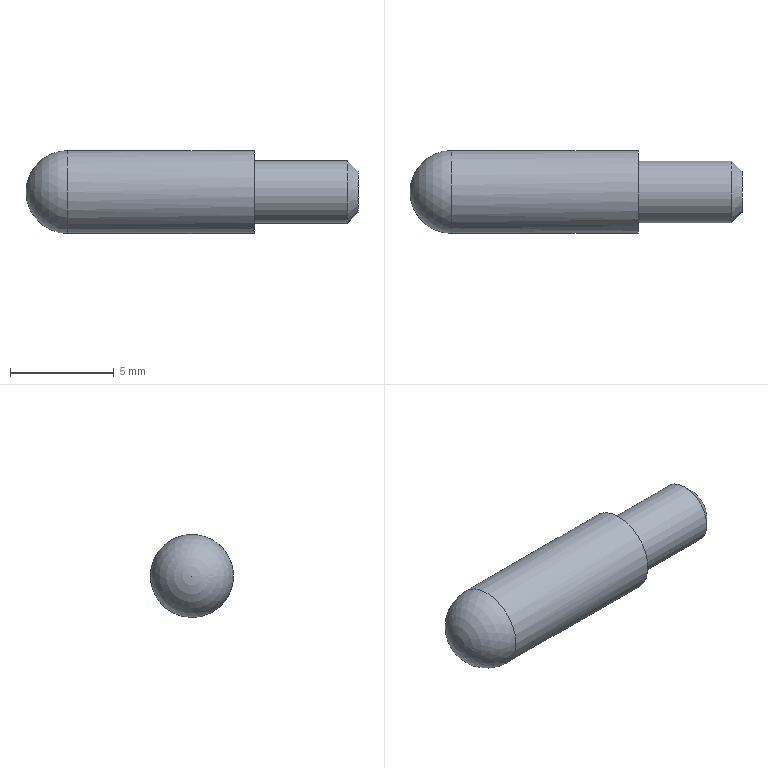Component | NX | ASSY_PRAC_PART_7 | 1 solid | 6 faces | box 16 x 4 x 4 mm | volume 164 mm3 | cylinder 2 | plane 2 | sphere 1 | cone 1 | commonest cylinder face diameters 4 x1 3 x1
STEP:
#1=CARTESIAN_POINT('',(0.,0.,0.));
#2=DIRECTION('',(0.,0.,1.));
#3=DIRECTION('',(1.,0.,0.));
#4=AXIS2_PLACEMENT_3D('',#1,#2,#3);
#5=CARTESIAN_POINT('',(-22.5,0.3851,13.561));
#6=VERTEX_POINT('',#5);
#7=CARTESIAN_POINT('',(-22.5,-1.615,15.561));
#8=VERTEX_POINT('',#7);
#9=CARTESIAN_POINT('',(-22.5,0.3851,15.561));
#10=DIRECTION('',(-1.,0.,0.));
#11=DIRECTION('',(0.,0.,-1.));
#12=AXIS2_PLACEMENT_3D('',#9,#10,#11);
#13=CIRCLE('',#12,2.);
#14=CARTESIAN_POINT('',(-22.5,0.3851,15.561));
#15=DIRECTION('',(-1.,-0.,0.));
#16=DIRECTION('',(0.,-1.,0.));
#17=AXIS2_PLACEMENT_3D('',#14,#15,#16);
#18=SPHERICAL_SURFACE('',#17,2.);
#19=CARTESIAN_POINT('',(4.712,0.));
#20=CARTESIAN_POINT('',(4.808,0.));
#21=CARTESIAN_POINT('',(4.998,0.));
#22=CARTESIAN_POINT('',(5.284,0.));
#23=CARTESIAN_POINT('',(5.569,0.));
#24=CARTESIAN_POINT('',(5.855,0.));
#25=CARTESIAN_POINT('',(6.14,0.));
#26=CARTESIAN_POINT('',(6.426,0.));
#27=CARTESIAN_POINT('',(6.712,0.));
#28=CARTESIAN_POINT('',(6.997,0.));
#29=CARTESIAN_POINT('',(7.283,0.));
#30=CARTESIAN_POINT('',(7.568,0.));
#31=CARTESIAN_POINT('',(7.854,0.));
#32=CARTESIAN_POINT('',(8.14,0.));
#33=CARTESIAN_POINT('',(8.425,0.));
#34=CARTESIAN_POINT('',(8.711,0.));
#35=CARTESIAN_POINT('',(8.996,0.));
#36=CARTESIAN_POINT('',(9.282,0.));
#37=CARTESIAN_POINT('',(9.568,0.));
#38=CARTESIAN_POINT('',(9.853,0.));
#39=CARTESIAN_POINT('',(10.139,0.));
#40=CARTESIAN_POINT('',(10.424,0.));
#41=CARTESIAN_POINT('',(10.71,0.));
#42=CARTESIAN_POINT('',(10.9,0.));
#43=CARTESIAN_POINT('',(10.996,0.));
#44=B_SPLINE_CURVE_WITH_KNOTS('',3,(#19,#20,#21,#22,#23,#24,#25,#26,#27,#28,#29,#30,#31,#32,#33,#34,#35,#36,#37,#38,#39,#40,#41,#42,#43),.UNSPECIFIED.,.F.,.F.,(4,1,1,1,1,1,1,1,1,1,1,1,1,1,1,1,1,1,1,1,1,1,4),(0.,0.2856,0.5712,0.8568,1.142,1.428,1.714,1.999,2.285,2.57,2.856,3.142,3.427,3.713,3.998,4.284,4.57,4.855,5.141,5.426,5.712,5.998,6.283),.QUASI_UNIFORM_KNOTS.);
#45=(GEOMETRIC_REPRESENTATION_CONTEXT(2)PARAMETRIC_REPRESENTATION_CONTEXT()REPRESENTATION_CONTEXT('',''));
#46=DEFINITIONAL_REPRESENTATION('',(#44),#45);
#47=PCURVE('',#18,#46);
#48=CARTESIAN_POINT('',(-24.5,0.3851,15.561));
#49=DIRECTION('',(-1.,0.,0.));
#50=DIRECTION('',(0.,0.,-1.));
#51=AXIS2_PLACEMENT_3D('',#48,#49,#50);
#52=CYLINDRICAL_SURFACE('',#51,2.);
#53=CARTESIAN_POINT('',(0.,-2.));
#54=DIRECTION('',(1.,0.));
#55=VECTOR('',#54,1.);
#56=LINE('',#53,#55);
#57=(GEOMETRIC_REPRESENTATION_CONTEXT(2)PARAMETRIC_REPRESENTATION_CONTEXT()REPRESENTATION_CONTEXT('',''));
#58=DEFINITIONAL_REPRESENTATION('',(#56),#57);
#59=PCURVE('',#52,#58);
#60=SURFACE_CURVE('',#13,(#47,#59),.PCURVE_S1.);
#61=EDGE_CURVE('',#6,#8,#60,.T.);
#62=ORIENTED_EDGE('',*,*,#61,.T.);
#63=CARTESIAN_POINT('',(-24.5,0.3851,15.561));
#64=VERTEX_POINT('',#63);
#65=CARTESIAN_POINT('',(-22.5,-1.615,15.561));
#66=CARTESIAN_POINT('',(-23.024,-1.615,15.561));
#67=CARTESIAN_POINT('',(-23.547,-1.45,15.561));
#68=CARTESIAN_POINT('',(-24.006,-1.121,15.561));
#69=CARTESIAN_POINT('',(-24.336,-0.6621,15.561));
#70=CARTESIAN_POINT('',(-24.5,-0.1385,15.561));
#71=CARTESIAN_POINT('',(-24.5,0.3851,15.561));
#72=B_SPLINE_CURVE_WITH_KNOTS('',6,(#65,#66,#67,#68,#69,#70,#71),.UNSPECIFIED.,.F.,.F.,(7,7),(0.,1.571),.PIECEWISE_BEZIER_KNOTS.);
#73=CARTESIAN_POINT('',(6.283,0.));
#74=DIRECTION('',(0.,1.));
#75=VECTOR('',#74,1.);
#76=LINE('',#73,#75);
#77=(GEOMETRIC_REPRESENTATION_CONTEXT(2)PARAMETRIC_REPRESENTATION_CONTEXT()REPRESENTATION_CONTEXT('',''));
#78=DEFINITIONAL_REPRESENTATION('',(#76),#77);
#79=PCURVE('',#18,#78);
#80=CARTESIAN_POINT('',(0.,0.));
#81=DIRECTION('',(0.,1.));
#82=VECTOR('',#81,1.);
#83=LINE('',#80,#82);
#84=(GEOMETRIC_REPRESENTATION_CONTEXT(2)PARAMETRIC_REPRESENTATION_CONTEXT()REPRESENTATION_CONTEXT('',''));
#85=DEFINITIONAL_REPRESENTATION('',(#83),#84);
#86=PCURVE('',#18,#85);
#87=SEAM_CURVE('',#72,(#79,#86),.PCURVE_S1.);
#88=EDGE_CURVE('',#8,#64,#87,.T.);
#89=ORIENTED_EDGE('',*,*,#88,.T.);
#90=ORIENTED_EDGE('',*,*,#88,.F.);
#91=CARTESIAN_POINT('',(-22.5,0.3851,15.561));
#92=DIRECTION('',(-1.,0.,0.));
#93=DIRECTION('',(0.,0.,-1.));
#94=AXIS2_PLACEMENT_3D('',#91,#92,#93);
#95=CIRCLE('',#94,2.);
#96=CARTESIAN_POINT('',(-1.571,0.));
#97=CARTESIAN_POINT('',(-1.476,0.));
#98=CARTESIAN_POINT('',(-1.285,0.));
#99=CARTESIAN_POINT('',(-0.9996,0.));
#100=CARTESIAN_POINT('',(-0.714,0.));
#101=CARTESIAN_POINT('',(-0.4284,0.));
#102=CARTESIAN_POINT('',(-0.1428,0.));
#103=CARTESIAN_POINT('',(0.1428,0.));
#104=CARTESIAN_POINT('',(0.4284,0.));
#105=CARTESIAN_POINT('',(0.714,0.));
#106=CARTESIAN_POINT('',(0.9996,0.));
#107=CARTESIAN_POINT('',(1.285,0.));
#108=CARTESIAN_POINT('',(1.571,0.));
#109=CARTESIAN_POINT('',(1.856,0.));
#110=CARTESIAN_POINT('',(2.142,0.));
#111=CARTESIAN_POINT('',(2.428,0.));
#112=CARTESIAN_POINT('',(2.713,0.));
#113=CARTESIAN_POINT('',(2.999,0.));
#114=CARTESIAN_POINT('',(3.284,0.));
#115=CARTESIAN_POINT('',(3.57,0.));
#116=CARTESIAN_POINT('',(3.856,0.));
#117=CARTESIAN_POINT('',(4.141,0.));
#118=CARTESIAN_POINT('',(4.427,0.));
#119=CARTESIAN_POINT('',(4.617,0.));
#120=CARTESIAN_POINT('',(4.712,0.));
#121=B_SPLINE_CURVE_WITH_KNOTS('',3,(#96,#97,#98,#99,#100,#101,#102,#103,#104,#105,#106,#107,#108,#109,#110,#111,#112,#113,#114,#115,#116,#117,#118,#119,#120),.UNSPECIFIED.,.F.,.F.,(4,1,1,1,1,1,1,1,1,1,1,1,1,1,1,1,1,1,1,1,1,1,4),(0.,0.2856,0.5712,0.8568,1.142,1.428,1.714,1.999,2.285,2.57,2.856,3.142,3.427,3.713,3.998,4.284,4.57,4.855,5.141,5.426,5.712,5.998,6.283),.QUASI_UNIFORM_KNOTS.);
#122=(GEOMETRIC_REPRESENTATION_CONTEXT(2)PARAMETRIC_REPRESENTATION_CONTEXT()REPRESENTATION_CONTEXT('',''));
#123=DEFINITIONAL_REPRESENTATION('',(#121),#122);
#124=PCURVE('',#18,#123);
#125=CARTESIAN_POINT('',(0.,-2.));
#126=DIRECTION('',(1.,0.));
#127=VECTOR('',#126,1.);
#128=LINE('',#125,#127);
#129=(GEOMETRIC_REPRESENTATION_CONTEXT(2)PARAMETRIC_REPRESENTATION_CONTEXT()REPRESENTATION_CONTEXT('',''));
#130=DEFINITIONAL_REPRESENTATION('',(#128),#129);
#131=PCURVE('',#52,#130);
#132=SURFACE_CURVE('',#95,(#124,#131),.PCURVE_S1.);
#133=EDGE_CURVE('',#8,#6,#132,.T.);
#134=ORIENTED_EDGE('',*,*,#133,.T.);
#135=EDGE_LOOP('',(#62,#89,#90,#134));
#136=FACE_BOUND('',#135,.T.);
#137=ADVANCED_FACE('',(#136),#18,.T.);
#138=ORIENTED_EDGE('',*,*,#61,.F.);
#139=CARTESIAN_POINT('',(-13.5,0.3851,13.561));
#140=VERTEX_POINT('',#139);
#141=CARTESIAN_POINT('',(-13.5,0.3851,13.561));
#142=CARTESIAN_POINT('',(-22.5,0.3851,13.561));
#143=B_SPLINE_CURVE_WITH_KNOTS('',1,(#141,#142),.UNSPECIFIED.,.F.,.F.,(2,2),(-11.,-2.),.PIECEWISE_BEZIER_KNOTS.);
#144=CARTESIAN_POINT('',(0.,0.));
#145=DIRECTION('',(0.,1.));
#146=VECTOR('',#145,1.);
#147=LINE('',#144,#146);
#148=(GEOMETRIC_REPRESENTATION_CONTEXT(2)PARAMETRIC_REPRESENTATION_CONTEXT()REPRESENTATION_CONTEXT('',''));
#149=DEFINITIONAL_REPRESENTATION('',(#147),#148);
#150=PCURVE('',#52,#149);
#151=CARTESIAN_POINT('',(6.283,0.));
#152=DIRECTION('',(0.,1.));
#153=VECTOR('',#152,1.);
#154=LINE('',#151,#153);
#155=(GEOMETRIC_REPRESENTATION_CONTEXT(2)PARAMETRIC_REPRESENTATION_CONTEXT()REPRESENTATION_CONTEXT('',''));
#156=DEFINITIONAL_REPRESENTATION('',(#154),#155);
#157=PCURVE('',#52,#156);
#158=SEAM_CURVE('',#143,(#150,#157),.PCURVE_S1.);
#159=EDGE_CURVE('',#140,#6,#158,.T.);
#160=ORIENTED_EDGE('',*,*,#159,.F.);
#161=CARTESIAN_POINT('',(-13.5,0.3851,15.561));
#162=DIRECTION('',(-1.,0.,0.));
#163=DIRECTION('',(0.,0.,-1.));
#164=AXIS2_PLACEMENT_3D('',#161,#162,#163);
#165=CIRCLE('',#164,2.);
#166=CARTESIAN_POINT('',(0.,-11.));
#167=DIRECTION('',(1.,0.));
#168=VECTOR('',#167,1.);
#169=LINE('',#166,#168);
#170=(GEOMETRIC_REPRESENTATION_CONTEXT(2)PARAMETRIC_REPRESENTATION_CONTEXT()REPRESENTATION_CONTEXT('',''));
#171=DEFINITIONAL_REPRESENTATION('',(#169),#170);
#172=PCURVE('',#52,#171);
#173=CARTESIAN_POINT('',(-13.5,-1.115,15.561));
#174=DIRECTION('',(-1.,0.,0.));
#175=DIRECTION('',(0.,0.,-1.));
#176=AXIS2_PLACEMENT_3D('',#173,#174,#175);
#177=PLANE('',#176);
#178=CARTESIAN_POINT('',(0.,-1.5));
#179=DIRECTION('',(1.,0.));
#180=AXIS2_PLACEMENT_2D('',#178,#179);
#181=CIRCLE('',#180,2.);
#182=(GEOMETRIC_REPRESENTATION_CONTEXT(2)PARAMETRIC_REPRESENTATION_CONTEXT()REPRESENTATION_CONTEXT('',''));
#183=DEFINITIONAL_REPRESENTATION('',(#181),#182);
#184=PCURVE('',#177,#183);
#185=SURFACE_CURVE('',#165,(#172,#184),.PCURVE_S1.);
#186=EDGE_CURVE('',#140,#140,#185,.T.);
#187=ORIENTED_EDGE('',*,*,#186,.T.);
#188=ORIENTED_EDGE('',*,*,#159,.T.);
#189=ORIENTED_EDGE('',*,*,#133,.F.);
#190=EDGE_LOOP('',(#138,#160,#187,#188,#189));
#191=FACE_BOUND('',#190,.T.);
#192=ADVANCED_FACE('',(#191),#52,.T.);
#193=ORIENTED_EDGE('',*,*,#186,.F.);
#194=EDGE_LOOP('',(#193));
#195=FACE_BOUND('',#194,.T.);
#196=CARTESIAN_POINT('',(-13.5,0.3851,14.061));
#197=VERTEX_POINT('',#196);
#198=CARTESIAN_POINT('',(-13.5,0.3851,15.561));
#199=DIRECTION('',(-1.,0.,0.));
#200=DIRECTION('',(0.,0.,-1.));
#201=AXIS2_PLACEMENT_3D('',#198,#199,#200);
#202=CIRCLE('',#201,1.5);
#203=CARTESIAN_POINT('',(0.,-1.5));
#204=DIRECTION('',(1.,0.));
#205=AXIS2_PLACEMENT_2D('',#203,#204);
#206=CIRCLE('',#205,1.5);
#207=(GEOMETRIC_REPRESENTATION_CONTEXT(2)PARAMETRIC_REPRESENTATION_CONTEXT()REPRESENTATION_CONTEXT('',''));
#208=DEFINITIONAL_REPRESENTATION('',(#206),#207);
#209=PCURVE('',#177,#208);
#210=CARTESIAN_POINT('',(-24.5,0.3851,15.561));
#211=DIRECTION('',(-1.,0.,0.));
#212=DIRECTION('',(0.,0.,-1.));
#213=AXIS2_PLACEMENT_3D('',#210,#211,#212);
#214=CYLINDRICAL_SURFACE('',#213,1.5);
#215=CARTESIAN_POINT('',(0.,-11.));
#216=DIRECTION('',(1.,0.));
#217=VECTOR('',#216,1.);
#218=LINE('',#215,#217);
#219=(GEOMETRIC_REPRESENTATION_CONTEXT(2)PARAMETRIC_REPRESENTATION_CONTEXT()REPRESENTATION_CONTEXT('',''));
#220=DEFINITIONAL_REPRESENTATION('',(#218),#219);
#221=PCURVE('',#214,#220);
#222=SURFACE_CURVE('',#202,(#209,#221),.PCURVE_S1.);
#223=EDGE_CURVE('',#197,#197,#222,.T.);
#224=ORIENTED_EDGE('',*,*,#223,.T.);
#225=EDGE_LOOP('',(#224));
#226=FACE_BOUND('',#225,.T.);
#227=ADVANCED_FACE('',(#195,#226),#177,.F.);
#228=CARTESIAN_POINT('',(-9.,0.3851,14.061));
#229=VERTEX_POINT('',#228);
#230=CARTESIAN_POINT('',(-9.,0.3851,15.561));
#231=DIRECTION('',(-1.,0.,0.));
#232=DIRECTION('',(0.,0.,-1.));
#233=AXIS2_PLACEMENT_3D('',#230,#231,#232);
#234=CIRCLE('',#233,1.5);
#235=CARTESIAN_POINT('',(0.,-15.5));
#236=DIRECTION('',(1.,0.));
#237=VECTOR('',#236,1.);
#238=LINE('',#235,#237);
#239=(GEOMETRIC_REPRESENTATION_CONTEXT(2)PARAMETRIC_REPRESENTATION_CONTEXT()REPRESENTATION_CONTEXT('',''));
#240=DEFINITIONAL_REPRESENTATION('',(#238),#239);
#241=PCURVE('',#214,#240);
#242=CARTESIAN_POINT('',(-9.,0.3851,15.561));
#243=DIRECTION('',(-1.,0.,0.));
#244=DIRECTION('',(0.,0.,-1.));
#245=AXIS2_PLACEMENT_3D('',#242,#243,#244);
#246=CONICAL_SURFACE('',#245,1.5,0.7854);
#247=CARTESIAN_POINT('',(0.,0.));
#248=DIRECTION('',(1.,0.));
#249=VECTOR('',#248,1.);
#250=LINE('',#247,#249);
#251=(GEOMETRIC_REPRESENTATION_CONTEXT(2)PARAMETRIC_REPRESENTATION_CONTEXT()REPRESENTATION_CONTEXT('',''));
#252=DEFINITIONAL_REPRESENTATION('',(#250),#251);
#253=PCURVE('',#246,#252);
#254=SURFACE_CURVE('',#234,(#241,#253),.PCURVE_S1.);
#255=EDGE_CURVE('',#229,#229,#254,.T.);
#256=ORIENTED_EDGE('',*,*,#255,.T.);
#257=CARTESIAN_POINT('',(-9.,0.3851,14.061));
#258=CARTESIAN_POINT('',(-13.5,0.3851,14.061));
#259=B_SPLINE_CURVE_WITH_KNOTS('',1,(#257,#258),.UNSPECIFIED.,.F.,.F.,(2,2),(-15.5,-11.),.PIECEWISE_BEZIER_KNOTS.);
#260=CARTESIAN_POINT('',(6.283,0.));
#261=DIRECTION('',(0.,1.));
#262=VECTOR('',#261,1.);
#263=LINE('',#260,#262);
#264=(GEOMETRIC_REPRESENTATION_CONTEXT(2)PARAMETRIC_REPRESENTATION_CONTEXT()REPRESENTATION_CONTEXT('',''));
#265=DEFINITIONAL_REPRESENTATION('',(#263),#264);
#266=PCURVE('',#214,#265);
#267=CARTESIAN_POINT('',(0.,0.));
#268=DIRECTION('',(0.,1.));
#269=VECTOR('',#268,1.);
#270=LINE('',#267,#269);
#271=(GEOMETRIC_REPRESENTATION_CONTEXT(2)PARAMETRIC_REPRESENTATION_CONTEXT()REPRESENTATION_CONTEXT('',''));
#272=DEFINITIONAL_REPRESENTATION('',(#270),#271);
#273=PCURVE('',#214,#272);
#274=SEAM_CURVE('',#259,(#266,#273),.PCURVE_S1.);
#275=EDGE_CURVE('',#229,#197,#274,.T.);
#276=ORIENTED_EDGE('',*,*,#275,.T.);
#277=ORIENTED_EDGE('',*,*,#223,.F.);
#278=ORIENTED_EDGE('',*,*,#275,.F.);
#279=EDGE_LOOP('',(#256,#276,#277,#278));
#280=FACE_BOUND('',#279,.T.);
#281=ADVANCED_FACE('',(#280),#214,.T.);
#282=CARTESIAN_POINT('',(-8.5,0.3851,14.561));
#283=VERTEX_POINT('',#282);
#284=CARTESIAN_POINT('',(-8.5,0.3851,15.561));
#285=DIRECTION('',(1.,0.,0.));
#286=DIRECTION('',(0.,0.,-1.));
#287=AXIS2_PLACEMENT_3D('',#284,#285,#286);
#288=CIRCLE('',#287,1.);
#289=CARTESIAN_POINT('',(-8.5,0.3851,15.561));
#290=DIRECTION('',(-1.,0.,0.));
#291=DIRECTION('',(0.,0.,-1.));
#292=AXIS2_PLACEMENT_3D('',#289,#290,#291);
#293=PLANE('',#292);
#294=CARTESIAN_POINT('',(1.,0.));
#295=CARTESIAN_POINT('',(1.,-1.732));
#296=CARTESIAN_POINT('',(-0.5,-0.866));
#297=CARTESIAN_POINT('',(-2.,-0.));
#298=CARTESIAN_POINT('',(-0.5,0.866));
#299=CARTESIAN_POINT('',(1.,1.732));
#300=CARTESIAN_POINT('',(1.,0.));
#301=(BOUNDED_CURVE()B_SPLINE_CURVE(2,(#294,#295,#296,#297,#298,#299,#300),.UNSPECIFIED.,.T.,.F.)B_SPLINE_CURVE_WITH_KNOTS((1,2,2,2,2,1),(-2.094,0.,2.094,4.189,6.283,8.378),.UNSPECIFIED.)CURVE()GEOMETRIC_REPRESENTATION_ITEM()RATIONAL_B_SPLINE_CURVE((1.,0.5,1.,0.5,1.,0.5,1.))REPRESENTATION_ITEM(''));
#302=(GEOMETRIC_REPRESENTATION_CONTEXT(2)PARAMETRIC_REPRESENTATION_CONTEXT()REPRESENTATION_CONTEXT('',''));
#303=DEFINITIONAL_REPRESENTATION('',(#301),#302);
#304=PCURVE('',#293,#303);
#305=CARTESIAN_POINT('',(6.283,-0.5));
#306=DIRECTION('',(-1.,0.));
#307=VECTOR('',#306,1.);
#308=LINE('',#305,#307);
#309=(GEOMETRIC_REPRESENTATION_CONTEXT(2)PARAMETRIC_REPRESENTATION_CONTEXT()REPRESENTATION_CONTEXT('',''));
#310=DEFINITIONAL_REPRESENTATION('',(#308),#309);
#311=PCURVE('',#246,#310);
#312=SURFACE_CURVE('',#288,(#304,#311),.PCURVE_S1.);
#313=EDGE_CURVE('',#283,#283,#312,.T.);
#314=ORIENTED_EDGE('',*,*,#313,.T.);
#315=EDGE_LOOP('',(#314));
#316=FACE_BOUND('',#315,.T.);
#317=ADVANCED_FACE('',(#316),#293,.F.);
#318=ORIENTED_EDGE('',*,*,#313,.F.);
#319=CARTESIAN_POINT('',(-8.5,0.3851,14.561));
#320=CARTESIAN_POINT('',(-9.,0.3851,14.061));
#321=B_SPLINE_CURVE_WITH_KNOTS('',1,(#319,#320),.UNSPECIFIED.,.F.,.F.,(2,2),(-0.7071,0.),.PIECEWISE_BEZIER_KNOTS.);
#322=CARTESIAN_POINT('',(6.283,0.));
#323=DIRECTION('',(0.,1.));
#324=VECTOR('',#323,1.);
#325=LINE('',#322,#324);
#326=(GEOMETRIC_REPRESENTATION_CONTEXT(2)PARAMETRIC_REPRESENTATION_CONTEXT()REPRESENTATION_CONTEXT('',''));
#327=DEFINITIONAL_REPRESENTATION('',(#325),#326);
#328=PCURVE('',#246,#327);
#329=CARTESIAN_POINT('',(0.,0.));
#330=DIRECTION('',(0.,1.));
#331=VECTOR('',#330,1.);
#332=LINE('',#329,#331);
#333=(GEOMETRIC_REPRESENTATION_CONTEXT(2)PARAMETRIC_REPRESENTATION_CONTEXT()REPRESENTATION_CONTEXT('',''));
#334=DEFINITIONAL_REPRESENTATION('',(#332),#333);
#335=PCURVE('',#246,#334);
#336=SEAM_CURVE('',#321,(#328,#335),.PCURVE_S1.);
#337=EDGE_CURVE('',#283,#229,#336,.T.);
#338=ORIENTED_EDGE('',*,*,#337,.T.);
#339=ORIENTED_EDGE('',*,*,#255,.F.);
#340=ORIENTED_EDGE('',*,*,#337,.F.);
#341=EDGE_LOOP('',(#318,#338,#339,#340));
#342=FACE_BOUND('',#341,.T.);
#343=ADVANCED_FACE('',(#342),#246,.T.);
#344=CLOSED_SHELL('',(#137,#192,#227,#281,#317,#343));
#345=MANIFOLD_SOLID_BREP('',#344);
#346=(LENGTH_UNIT()NAMED_UNIT(*)SI_UNIT(.MILLI.,.METRE.));
#347=UNCERTAINTY_MEASURE_WITH_UNIT(LENGTH_MEASURE(0.00001),#346,'','');
#348=(NAMED_UNIT(*)PLANE_ANGLE_UNIT()SI_UNIT($,.RADIAN.));
#349=(NAMED_UNIT(*)SI_UNIT($,.STERADIAN.)SOLID_ANGLE_UNIT());
#350=(GEOMETRIC_REPRESENTATION_CONTEXT(3)GLOBAL_UNCERTAINTY_ASSIGNED_CONTEXT((#347))GLOBAL_UNIT_ASSIGNED_CONTEXT((#346,#348,#349))REPRESENTATION_CONTEXT('',''));
#351=ADVANCED_BREP_SHAPE_REPRESENTATION('',(#4,#345),#350);